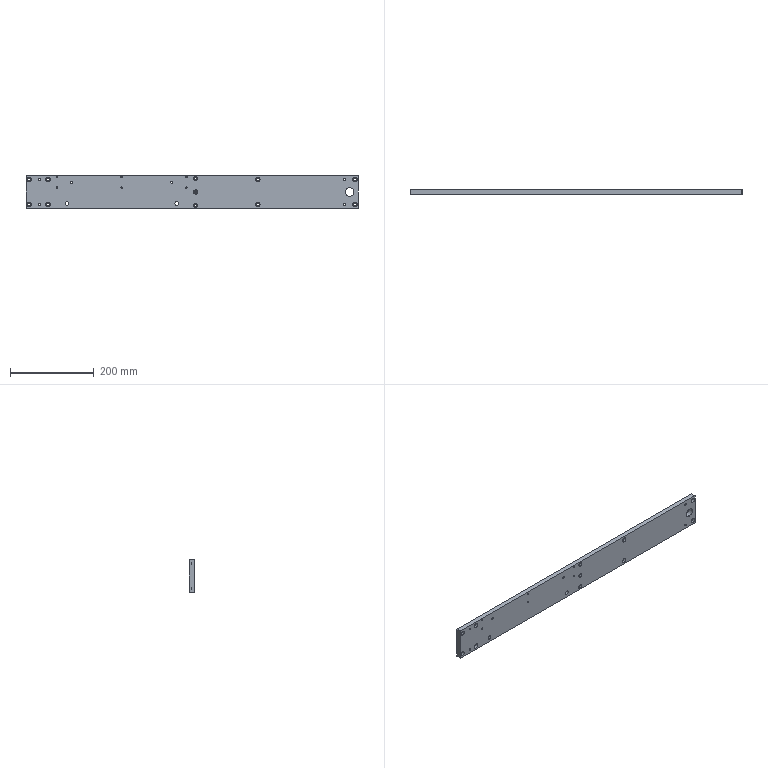Component | SolidWorks | A066-2 | 1 solid | 95 faces | box 795 x 12 x 80 mm | volume 747834 mm3 | cylinder 74 | plane 21 | commonest cylinder face diameters 11 x16 6.4 x16 5 x12 3.3 x12 10 x6 5.3 x6 9 x4 20 x2
build123d program:
from build123d import *

# Parameters (mm, degrees)
SKETCH1_W                                       = 80
SKETCH1_H                                       = 795
BOSS_EXTRUDE1_DEPTH                             = 12
M6_HEX_SOCKET_HEAD_CAP_SCREW_CBORE1_D           = 6.4
M6_HEX_SOCKET_HEAD_CAP_SCREW_CBORE1_CBORE_D     = 11
M6_HEX_SOCKET_HEAD_CAP_SCREW_CBORE1_CBORE_DEPTH = 6.4
F_5_0_5_DIAMETER_HOLE1_D                        = 5
CHAMFER1_SIZE                                   = 1
M6_HEX_SOCKET_HEAD_CAP_SCREW_CBORE2_D           = 6.4
M6_HEX_SOCKET_HEAD_CAP_SCREW_CBORE2_CBORE_D     = 11
M6_HEX_SOCKET_HEAD_CAP_SCREW_CBORE2_CBORE_DEPTH = 6.4
SKETCH8_R                                       = 10
CUT_EXTRUDE1_DEPTH                              = 400.688
M5_HEX_SOCKET_HEAD_CAP_SCREW_CBORE1_D           = 5.3
M5_HEX_SOCKET_HEAD_CAP_SCREW_CBORE1_CBORE_D     = 10
M5_HEX_SOCKET_HEAD_CAP_SCREW_CBORE1_CBORE_DEPTH = 5.4
M4_TAPPED_HOLE1_D                               = 3.3
F_5_0_5_DIAMETER_HOLE2_D                        = 5
M10X1_0_TAPPED_HOLE1_D                          = 9


with BuildPart() as part:
    # Sketch1 → Boss-Extrude1 (new body)
    with BuildSketch(Plane.XY):
        Rectangle(SKETCH1_W, SKETCH1_H)
    extrude(amount=BOSS_EXTRUDE1_DEPTH)

    # M6 Hex Socket Head Cap Screw CBORE1 (through all)
    with Locations(Plane.XY.offset(12)):
        with Locations((30, 390), (-30, 390), (30, -390), (-30, -390)):
            CounterBoreHole(M6_HEX_SOCKET_HEAD_CAP_SCREW_CBORE1_D / 2, M6_HEX_SOCKET_HEAD_CAP_SCREW_CBORE1_CBORE_D / 2, M6_HEX_SOCKET_HEAD_CAP_SCREW_CBORE1_CBORE_DEPTH)

    # 5.0 _5_ Diameter Hole1 (through all)
    with Locations(Plane(origin=(0, 0, 0), x_dir=(-1, 0, 0), z_dir=(0, 0, -1))):
        with Locations((-30, -365), (30, -365), (-30, 365), (30, 365)):
            Hole(F_5_0_5_DIAMETER_HOLE1_D / 2)

    # Chamfer1
    chamfer1_edges = [part.edges().sort_by_distance(p)[0] for p in [
        (40, -397.5, 6),
        (-40, -397.5, 6),
        (-40, 397.5, 6),
        (40, 397.5, 6),
    ]]
    chamfer(chamfer1_edges, length=CHAMFER1_SIZE)

    # M6 Hex Socket Head Cap Screw CBORE2 (through all)
    with Locations(Plane.XY.offset(12)):
        with Locations((-30, -344.5), (30, -344.5), (-30, 157.5), (30, 157.5)):
            CounterBoreHole(M6_HEX_SOCKET_HEAD_CAP_SCREW_CBORE2_D / 2, M6_HEX_SOCKET_HEAD_CAP_SCREW_CBORE2_CBORE_D / 2, M6_HEX_SOCKET_HEAD_CAP_SCREW_CBORE2_CBORE_DEPTH)

    # Sketch8 → Cut-Extrude1 (cut, through all)
    with BuildSketch(Plane.XY.offset(12)):
        with Locations((0, 377.5)):
            Circle(SKETCH8_R)
    extrude(amount=-CUT_EXTRUDE1_DEPTH, mode=Mode.SUBTRACT)

    # M5 Hex Socket Head Cap Screw CBORE1 (through all)
    with Locations(Plane.XY.offset(12)):
        with Locations((32.5, 8.5), (0, 8.5), (-32.5, 8.5)):
            CounterBoreHole(M5_HEX_SOCKET_HEAD_CAP_SCREW_CBORE1_D / 2, M5_HEX_SOCKET_HEAD_CAP_SCREW_CBORE1_CBORE_D / 2, M5_HEX_SOCKET_HEAD_CAP_SCREW_CBORE1_CBORE_DEPTH)

    # M4 Tapped Hole1 (through all)
    with Locations(Plane(origin=(0, 0, 0), x_dir=(-1, 0, 0), z_dir=(0, 0, -1))):
        with Locations((35.5, -13.5), (10.5, -13.5), (35.5, -168.5), (10.5, -168.5), (35.5, -323.5), (10.5, -323.5)):
            Hole(M4_TAPPED_HOLE1_D / 2)

    # 5.0 _5_ Diameter Hole2 (through all)
    with Locations(Plane(origin=(0, 0, 0), x_dir=(-1, 0, 0), z_dir=(0, 0, -1))):
        with Locations((23, -48.5), (23, -288.5)):
            Hole(F_5_0_5_DIAMETER_HOLE2_D / 2)

    # M10x1.0 Tapped Hole1 (through all)
    with Locations(Plane.XY.offset(12)):
        with Locations((27.5, -299.5), (27.5, -36.5)):
            Hole(M10X1_0_TAPPED_HOLE1_D / 2)


solid = part.part

# Placed as in the assembly
solid = solid.moved(Location((318.881, 0, 60), (90, 0, -90)))